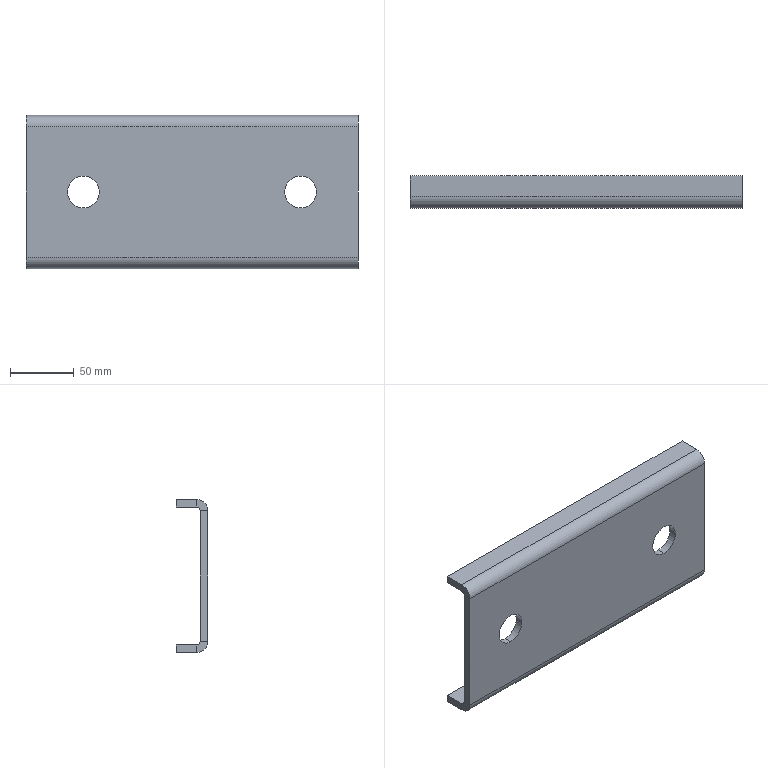Component | SolidWorks | THK-A1018FrontGuideWheelMountingPlate-1 | 1 solid | 26 faces | box 260 x 25 x 120 mm | volume 232555 mm3 | plane 18 | cylinder 8 | commonest cylinder face diameters 25 x4 18 x2 6 x2 | material Q235A
STEP:
#1=CARTESIAN_POINT('',(3.346,-5.079,-46.004));
#2=VERTEX_POINT('',#1);
#3=CARTESIAN_POINT('',(3.346,-5.079,-46.988));
#4=VERTEX_POINT('',#3);
#5=CARTESIAN_POINT('',(3.346,-5.079,-46.496));
#6=DIRECTION('',(0.,-1.,0.));
#7=DIRECTION('',(0.,0.,-1.));
#8=AXIS2_PLACEMENT_3D('',#5,#6,#7);
#9=CIRCLE('',#8,0.4921);
#10=EDGE_CURVE('',#2,#4,#9,.T.);
#11=ORIENTED_EDGE('',*,*,#10,.F.);
#12=CARTESIAN_POINT('',(3.346,-5.315,-46.004));
#13=VERTEX_POINT('',#12);
#14=CARTESIAN_POINT('',(3.346,-5.315,-46.004));
#15=DIRECTION('',(0.,-1.,0.));
#16=VECTOR('',#15,39.37);
#17=LINE('',#14,#16);
#18=EDGE_CURVE('',#2,#13,#17,.T.);
#19=ORIENTED_EDGE('',*,*,#18,.T.);
#20=CARTESIAN_POINT('',(3.346,-5.315,-46.988));
#21=VERTEX_POINT('',#20);
#22=CARTESIAN_POINT('',(3.346,-5.315,-46.496));
#23=DIRECTION('',(0.,-1.,0.));
#24=DIRECTION('',(0.,0.,-1.));
#25=AXIS2_PLACEMENT_3D('',#22,#23,#24);
#26=CIRCLE('',#25,0.4921);
#27=EDGE_CURVE('',#13,#21,#26,.T.);
#28=ORIENTED_EDGE('',*,*,#27,.T.);
#29=CARTESIAN_POINT('',(3.346,-5.315,-46.988));
#30=DIRECTION('',(0.,-1.,0.));
#31=VECTOR('',#30,39.37);
#32=LINE('',#29,#31);
#33=EDGE_CURVE('',#4,#21,#32,.T.);
#34=ORIENTED_EDGE('',*,*,#33,.F.);
#35=EDGE_LOOP('',(#11,#19,#28,#34));
#36=FACE_OUTER_BOUND('',#35,.T.);
#37=CARTESIAN_POINT('',(3.346,-5.315,-46.496));
#38=DIRECTION('',(0.,-1.,0.));
#39=DIRECTION('',(0.,0.,-1.));
#40=AXIS2_PLACEMENT_3D('',#37,#38,#39);
#41=CYLINDRICAL_SURFACE('',#40,0.4921);
#42=ADVANCED_FACE('',(#36),#41,.F.);
#43=CARTESIAN_POINT('',(-3.346,-5.079,-46.004));
#44=VERTEX_POINT('',#43);
#45=CARTESIAN_POINT('',(-3.346,-5.079,-46.988));
#46=VERTEX_POINT('',#45);
#47=CARTESIAN_POINT('',(-3.346,-5.079,-46.496));
#48=DIRECTION('',(0.,-1.,0.));
#49=DIRECTION('',(0.,0.,-1.));
#50=AXIS2_PLACEMENT_3D('',#47,#48,#49);
#51=CIRCLE('',#50,0.4921);
#52=EDGE_CURVE('',#44,#46,#51,.T.);
#53=ORIENTED_EDGE('',*,*,#52,.F.);
#54=CARTESIAN_POINT('',(-3.346,-5.315,-46.004));
#55=VERTEX_POINT('',#54);
#56=CARTESIAN_POINT('',(-3.346,-5.315,-46.004));
#57=DIRECTION('',(0.,-1.,0.));
#58=VECTOR('',#57,39.37);
#59=LINE('',#56,#58);
#60=EDGE_CURVE('',#44,#55,#59,.T.);
#61=ORIENTED_EDGE('',*,*,#60,.T.);
#62=CARTESIAN_POINT('',(-3.346,-5.315,-46.988));
#63=VERTEX_POINT('',#62);
#64=CARTESIAN_POINT('',(-3.346,-5.315,-46.496));
#65=DIRECTION('',(0.,-1.,0.));
#66=DIRECTION('',(0.,0.,-1.));
#67=AXIS2_PLACEMENT_3D('',#64,#65,#66);
#68=CIRCLE('',#67,0.4921);
#69=EDGE_CURVE('',#55,#63,#68,.T.);
#70=ORIENTED_EDGE('',*,*,#69,.T.);
#71=CARTESIAN_POINT('',(-3.346,-5.315,-46.988));
#72=DIRECTION('',(0.,-1.,0.));
#73=VECTOR('',#72,39.37);
#74=LINE('',#71,#73);
#75=EDGE_CURVE('',#46,#63,#74,.T.);
#76=ORIENTED_EDGE('',*,*,#75,.F.);
#77=EDGE_LOOP('',(#53,#61,#70,#76));
#78=FACE_OUTER_BOUND('',#77,.T.);
#79=CARTESIAN_POINT('',(-3.346,-5.315,-46.496));
#80=DIRECTION('',(0.,-1.,0.));
#81=DIRECTION('',(0.,0.,-1.));
#82=AXIS2_PLACEMENT_3D('',#79,#80,#81);
#83=CYLINDRICAL_SURFACE('',#82,0.4921);
#84=ADVANCED_FACE('',(#78),#83,.F.);
#85=CARTESIAN_POINT('',(5.118,-5.315,-48.504));
#86=VERTEX_POINT('',#85);
#87=CARTESIAN_POINT('',(5.118,-5.079,-48.504));
#88=VERTEX_POINT('',#87);
#89=CARTESIAN_POINT('',(5.118,-5.315,-48.504));
#90=DIRECTION('',(0.,1.,0.));
#91=VECTOR('',#90,39.37);
#92=LINE('',#89,#91);
#93=EDGE_CURVE('',#86,#88,#92,.T.);
#94=ORIENTED_EDGE('',*,*,#93,.F.);
#95=CARTESIAN_POINT('',(5.118,-4.961,-48.858));
#96=VERTEX_POINT('',#95);
#97=CARTESIAN_POINT('',(5.118,-4.961,-48.504));
#98=DIRECTION('',(-1.,0.,0.));
#99=DIRECTION('',(0.,0.,-1.));
#100=AXIS2_PLACEMENT_3D('',#97,#98,#99);
#101=CIRCLE('',#100,0.3543);
#102=EDGE_CURVE('',#96,#86,#101,.T.);
#103=ORIENTED_EDGE('',*,*,#102,.F.);
#104=CARTESIAN_POINT('',(5.118,-4.961,-48.622));
#105=VERTEX_POINT('',#104);
#106=CARTESIAN_POINT('',(5.118,-4.961,-48.622));
#107=DIRECTION('',(0.,0.,-1.));
#108=VECTOR('',#107,39.37);
#109=LINE('',#106,#108);
#110=EDGE_CURVE('',#105,#96,#109,.T.);
#111=ORIENTED_EDGE('',*,*,#110,.F.);
#112=CARTESIAN_POINT('',(5.118,-4.961,-48.504));
#113=DIRECTION('',(-1.,0.,0.));
#114=DIRECTION('',(0.,0.,-1.));
#115=AXIS2_PLACEMENT_3D('',#112,#113,#114);
#116=CIRCLE('',#115,0.1181);
#117=EDGE_CURVE('',#105,#88,#116,.T.);
#118=ORIENTED_EDGE('',*,*,#117,.T.);
#119=EDGE_LOOP('',(#94,#103,#111,#118));
#120=FACE_OUTER_BOUND('',#119,.T.);
#121=CARTESIAN_POINT('',(5.118,-5.315,-48.504));
#122=DIRECTION('',(1.,0.,0.));
#123=DIRECTION('',(0.,0.,-1.));
#124=AXIS2_PLACEMENT_3D('',#121,#122,#123);
#125=PLANE('',#124);
#126=ADVANCED_FACE('',(#120),#125,.T.);
#127=CARTESIAN_POINT('',(5.118,-5.315,-44.488));
#128=VERTEX_POINT('',#127);
#129=CARTESIAN_POINT('',(5.118,-5.315,-44.134));
#130=DIRECTION('',(0.,0.,1.));
#131=VECTOR('',#130,39.37);
#132=LINE('',#129,#131);
#133=EDGE_CURVE('',#86,#128,#132,.T.);
#134=ORIENTED_EDGE('',*,*,#133,.F.);
#135=ORIENTED_EDGE('',*,*,#93,.T.);
#136=CARTESIAN_POINT('',(5.118,-5.079,-44.488));
#137=VERTEX_POINT('',#136);
#138=CARTESIAN_POINT('',(5.118,-5.079,-44.134));
#139=DIRECTION('',(0.,0.,1.));
#140=VECTOR('',#139,39.37);
#141=LINE('',#138,#140);
#142=EDGE_CURVE('',#88,#137,#141,.T.);
#143=ORIENTED_EDGE('',*,*,#142,.T.);
#144=CARTESIAN_POINT('',(5.118,-5.079,-44.488));
#145=DIRECTION('',(0.,-1.,0.));
#146=VECTOR('',#145,39.37);
#147=LINE('',#144,#146);
#148=EDGE_CURVE('',#137,#128,#147,.T.);
#149=ORIENTED_EDGE('',*,*,#148,.T.);
#150=EDGE_LOOP('',(#134,#135,#143,#149));
#151=FACE_OUTER_BOUND('',#150,.T.);
#152=CARTESIAN_POINT('',(5.118,-4.961,-48.622));
#153=DIRECTION('',(1.,0.,0.));
#154=DIRECTION('',(0.,0.,-1.));
#155=AXIS2_PLACEMENT_3D('',#152,#153,#154);
#156=PLANE('',#155);
#157=ADVANCED_FACE('',(#151),#156,.T.);
#158=CARTESIAN_POINT('',(-5.118,-4.961,-48.858));
#159=VERTEX_POINT('',#158);
#160=CARTESIAN_POINT('',(-5.118,-4.961,-48.622));
#161=VERTEX_POINT('',#160);
#162=CARTESIAN_POINT('',(-5.118,-4.961,-48.858));
#163=DIRECTION('',(0.,0.,1.));
#164=VECTOR('',#163,39.37);
#165=LINE('',#162,#164);
#166=EDGE_CURVE('',#159,#161,#165,.T.);
#167=ORIENTED_EDGE('',*,*,#166,.F.);
#168=CARTESIAN_POINT('',(-5.118,-5.315,-48.504));
#169=VERTEX_POINT('',#168);
#170=CARTESIAN_POINT('',(-5.118,-4.961,-48.504));
#171=DIRECTION('',(-1.,0.,0.));
#172=DIRECTION('',(0.,0.,-1.));
#173=AXIS2_PLACEMENT_3D('',#170,#171,#172);
#174=CIRCLE('',#173,0.3543);
#175=EDGE_CURVE('',#159,#169,#174,.T.);
#176=ORIENTED_EDGE('',*,*,#175,.T.);
#177=CARTESIAN_POINT('',(-5.118,-5.079,-48.504));
#178=VERTEX_POINT('',#177);
#179=CARTESIAN_POINT('',(-5.118,-5.079,-48.504));
#180=DIRECTION('',(0.,-1.,0.));
#181=VECTOR('',#180,39.37);
#182=LINE('',#179,#181);
#183=EDGE_CURVE('',#178,#169,#182,.T.);
#184=ORIENTED_EDGE('',*,*,#183,.F.);
#185=CARTESIAN_POINT('',(-5.118,-4.961,-48.504));
#186=DIRECTION('',(-1.,0.,0.));
#187=DIRECTION('',(0.,0.,-1.));
#188=AXIS2_PLACEMENT_3D('',#185,#186,#187);
#189=CIRCLE('',#188,0.1181);
#190=EDGE_CURVE('',#161,#178,#189,.T.);
#191=ORIENTED_EDGE('',*,*,#190,.F.);
#192=EDGE_LOOP('',(#167,#176,#184,#191));
#193=FACE_OUTER_BOUND('',#192,.T.);
#194=CARTESIAN_POINT('',(-5.118,-4.961,-48.858));
#195=DIRECTION('',(-1.,0.,0.));
#196=DIRECTION('',(0.,0.,1.));
#197=AXIS2_PLACEMENT_3D('',#194,#195,#196);
#198=PLANE('',#197);
#199=ADVANCED_FACE('',(#193),#198,.T.);
#200=CARTESIAN_POINT('',(-5.118,-4.331,-48.858));
#201=VERTEX_POINT('',#200);
#202=CARTESIAN_POINT('',(-5.118,-5.315,-48.858));
#203=DIRECTION('',(0.,-1.,0.));
#204=VECTOR('',#203,39.37);
#205=LINE('',#202,#204);
#206=EDGE_CURVE('',#201,#159,#205,.T.);
#207=ORIENTED_EDGE('',*,*,#206,.T.);
#208=ORIENTED_EDGE('',*,*,#166,.T.);
#209=CARTESIAN_POINT('',(-5.118,-4.331,-48.622));
#210=VERTEX_POINT('',#209);
#211=CARTESIAN_POINT('',(-5.118,-5.315,-48.622));
#212=DIRECTION('',(0.,-1.,0.));
#213=VECTOR('',#212,39.37);
#214=LINE('',#211,#213);
#215=EDGE_CURVE('',#210,#161,#214,.T.);
#216=ORIENTED_EDGE('',*,*,#215,.F.);
#217=CARTESIAN_POINT('',(-5.118,-4.331,-48.622));
#218=DIRECTION('',(0.,0.,-1.));
#219=VECTOR('',#218,39.37);
#220=LINE('',#217,#219);
#221=EDGE_CURVE('',#210,#201,#220,.T.);
#222=ORIENTED_EDGE('',*,*,#221,.T.);
#223=EDGE_LOOP('',(#207,#208,#216,#222));
#224=FACE_OUTER_BOUND('',#223,.T.);
#225=CARTESIAN_POINT('',(-5.118,-5.079,-48.504));
#226=DIRECTION('',(-1.,0.,0.));
#227=DIRECTION('',(0.,0.,1.));
#228=AXIS2_PLACEMENT_3D('',#225,#226,#227);
#229=PLANE('',#228);
#230=ADVANCED_FACE('',(#224),#229,.T.);
#231=CARTESIAN_POINT('',(5.118,-4.961,-44.134));
#232=VERTEX_POINT('',#231);
#233=CARTESIAN_POINT('',(5.118,-4.961,-44.37));
#234=VERTEX_POINT('',#233);
#235=CARTESIAN_POINT('',(5.118,-4.961,-44.134));
#236=DIRECTION('',(0.,0.,-1.));
#237=VECTOR('',#236,39.37);
#238=LINE('',#235,#237);
#239=EDGE_CURVE('',#232,#234,#238,.T.);
#240=ORIENTED_EDGE('',*,*,#239,.F.);
#241=CARTESIAN_POINT('',(5.118,-4.961,-44.488));
#242=DIRECTION('',(-1.,0.,0.));
#243=DIRECTION('',(0.,0.,-1.));
#244=AXIS2_PLACEMENT_3D('',#241,#242,#243);
#245=CIRCLE('',#244,0.3543);
#246=EDGE_CURVE('',#128,#232,#245,.T.);
#247=ORIENTED_EDGE('',*,*,#246,.F.);
#248=ORIENTED_EDGE('',*,*,#148,.F.);
#249=CARTESIAN_POINT('',(5.118,-4.961,-44.488));
#250=DIRECTION('',(-1.,0.,0.));
#251=DIRECTION('',(0.,0.,-1.));
#252=AXIS2_PLACEMENT_3D('',#249,#250,#251);
#253=CIRCLE('',#252,0.1181);
#254=EDGE_CURVE('',#137,#234,#253,.T.);
#255=ORIENTED_EDGE('',*,*,#254,.T.);
#256=EDGE_LOOP('',(#240,#247,#248,#255));
#257=FACE_OUTER_BOUND('',#256,.T.);
#258=CARTESIAN_POINT('',(5.118,-4.961,-44.134));
#259=DIRECTION('',(1.,0.,0.));
#260=DIRECTION('',(0.,0.,-1.));
#261=AXIS2_PLACEMENT_3D('',#258,#259,#260);
#262=PLANE('',#261);
#263=ADVANCED_FACE('',(#257),#262,.T.);
#264=CARTESIAN_POINT('',(5.118,-4.331,-44.134));
#265=VERTEX_POINT('',#264);
#266=CARTESIAN_POINT('',(5.118,-5.315,-44.134));
#267=DIRECTION('',(0.,1.,0.));
#268=VECTOR('',#267,39.37);
#269=LINE('',#266,#268);
#270=EDGE_CURVE('',#232,#265,#269,.T.);
#271=ORIENTED_EDGE('',*,*,#270,.F.);
#272=ORIENTED_EDGE('',*,*,#239,.T.);
#273=CARTESIAN_POINT('',(5.118,-4.331,-44.37));
#274=VERTEX_POINT('',#273);
#275=CARTESIAN_POINT('',(5.118,-5.315,-44.37));
#276=DIRECTION('',(0.,1.,0.));
#277=VECTOR('',#276,39.37);
#278=LINE('',#275,#277);
#279=EDGE_CURVE('',#234,#274,#278,.T.);
#280=ORIENTED_EDGE('',*,*,#279,.T.);
#281=CARTESIAN_POINT('',(5.118,-4.331,-44.134));
#282=DIRECTION('',(0.,0.,-1.));
#283=VECTOR('',#282,39.37);
#284=LINE('',#281,#283);
#285=EDGE_CURVE('',#265,#274,#284,.T.);
#286=ORIENTED_EDGE('',*,*,#285,.F.);
#287=EDGE_LOOP('',(#271,#272,#280,#286));
#288=FACE_OUTER_BOUND('',#287,.T.);
#289=CARTESIAN_POINT('',(5.118,-5.079,-44.488));
#290=DIRECTION('',(1.,0.,0.));
#291=DIRECTION('',(0.,0.,-1.));
#292=AXIS2_PLACEMENT_3D('',#289,#290,#291);
#293=PLANE('',#292);
#294=ADVANCED_FACE('',(#288),#293,.T.);
#295=CARTESIAN_POINT('',(-5.118,-5.315,-44.488));
#296=VERTEX_POINT('',#295);
#297=CARTESIAN_POINT('',(-5.118,-5.079,-44.488));
#298=VERTEX_POINT('',#297);
#299=CARTESIAN_POINT('',(-5.118,-5.315,-44.488));
#300=DIRECTION('',(0.,1.,0.));
#301=VECTOR('',#300,39.37);
#302=LINE('',#299,#301);
#303=EDGE_CURVE('',#296,#298,#302,.T.);
#304=ORIENTED_EDGE('',*,*,#303,.F.);
#305=CARTESIAN_POINT('',(-5.118,-4.961,-44.134));
#306=VERTEX_POINT('',#305);
#307=CARTESIAN_POINT('',(-5.118,-4.961,-44.488));
#308=DIRECTION('',(-1.,0.,0.));
#309=DIRECTION('',(0.,0.,-1.));
#310=AXIS2_PLACEMENT_3D('',#307,#308,#309);
#311=CIRCLE('',#310,0.3543);
#312=EDGE_CURVE('',#296,#306,#311,.T.);
#313=ORIENTED_EDGE('',*,*,#312,.T.);
#314=CARTESIAN_POINT('',(-5.118,-4.961,-44.37));
#315=VERTEX_POINT('',#314);
#316=CARTESIAN_POINT('',(-5.118,-4.961,-44.37));
#317=DIRECTION('',(0.,0.,1.));
#318=VECTOR('',#317,39.37);
#319=LINE('',#316,#318);
#320=EDGE_CURVE('',#315,#306,#319,.T.);
#321=ORIENTED_EDGE('',*,*,#320,.F.);
#322=CARTESIAN_POINT('',(-5.118,-4.961,-44.488));
#323=DIRECTION('',(-1.,0.,0.));
#324=DIRECTION('',(0.,0.,-1.));
#325=AXIS2_PLACEMENT_3D('',#322,#323,#324);
#326=CIRCLE('',#325,0.1181);
#327=EDGE_CURVE('',#298,#315,#326,.T.);
#328=ORIENTED_EDGE('',*,*,#327,.F.);
#329=EDGE_LOOP('',(#304,#313,#321,#328));
#330=FACE_OUTER_BOUND('',#329,.T.);
#331=CARTESIAN_POINT('',(-5.118,-5.315,-44.488));
#332=DIRECTION('',(-1.,0.,0.));
#333=DIRECTION('',(0.,0.,1.));
#334=AXIS2_PLACEMENT_3D('',#331,#332,#333);
#335=PLANE('',#334);
#336=ADVANCED_FACE('',(#330),#335,.T.);
#337=CARTESIAN_POINT('',(-5.118,-5.315,-44.134));
#338=DIRECTION('',(0.,0.,1.));
#339=VECTOR('',#338,39.37);
#340=LINE('',#337,#339);
#341=EDGE_CURVE('',#169,#296,#340,.T.);
#342=ORIENTED_EDGE('',*,*,#341,.T.);
#343=ORIENTED_EDGE('',*,*,#303,.T.);
#344=CARTESIAN_POINT('',(-5.118,-5.079,-44.134));
#345=DIRECTION('',(0.,0.,1.));
#346=VECTOR('',#345,39.37);
#347=LINE('',#344,#346);
#348=EDGE_CURVE('',#178,#298,#347,.T.);
#349=ORIENTED_EDGE('',*,*,#348,.F.);
#350=ORIENTED_EDGE('',*,*,#183,.T.);
#351=EDGE_LOOP('',(#342,#343,#349,#350));
#352=FACE_OUTER_BOUND('',#351,.T.);
#353=CARTESIAN_POINT('',(-5.118,-4.961,-44.37));
#354=DIRECTION('',(-1.,0.,0.));
#355=DIRECTION('',(0.,0.,1.));
#356=AXIS2_PLACEMENT_3D('',#353,#354,#355);
#357=PLANE('',#356);
#358=ADVANCED_FACE('',(#352),#357,.T.);
#359=CARTESIAN_POINT('',(-5.118,-4.331,-44.37));
#360=VERTEX_POINT('',#359);
#361=CARTESIAN_POINT('',(-5.118,-5.315,-44.37));
#362=DIRECTION('',(0.,1.,0.));
#363=VECTOR('',#362,39.37);
#364=LINE('',#361,#363);
#365=EDGE_CURVE('',#315,#360,#364,.T.);
#366=ORIENTED_EDGE('',*,*,#365,.T.);
#367=CARTESIAN_POINT('',(5.118,-4.331,-44.37));
#368=DIRECTION('',(-1.,0.,0.));
#369=VECTOR('',#368,39.37);
#370=LINE('',#367,#369);
#371=EDGE_CURVE('',#274,#360,#370,.T.);
#372=ORIENTED_EDGE('',*,*,#371,.F.);
#373=ORIENTED_EDGE('',*,*,#279,.F.);
#374=CARTESIAN_POINT('',(5.118,-4.961,-44.37));
#375=DIRECTION('',(-1.,0.,0.));
#376=VECTOR('',#375,39.37);
#377=LINE('',#374,#376);
#378=EDGE_CURVE('',#234,#315,#377,.T.);
#379=ORIENTED_EDGE('',*,*,#378,.T.);
#380=EDGE_LOOP('',(#366,#372,#373,#379));
#381=FACE_OUTER_BOUND('',#380,.T.);
#382=CARTESIAN_POINT('',(5.118,-5.315,-44.37));
#383=DIRECTION('',(0.,0.,1.));
#384=DIRECTION('',(1.,0.,0.));
#385=AXIS2_PLACEMENT_3D('',#382,#383,#384);
#386=PLANE('',#385);
#387=ADVANCED_FACE('',(#381),#386,.F.);
#388=CARTESIAN_POINT('',(-5.118,-4.331,-44.134));
#389=VERTEX_POINT('',#388);
#390=CARTESIAN_POINT('',(-5.118,-4.331,-44.134));
#391=DIRECTION('',(0.,0.,-1.));
#392=VECTOR('',#391,39.37);
#393=LINE('',#390,#392);
#394=EDGE_CURVE('',#389,#360,#393,.T.);
#395=ORIENTED_EDGE('',*,*,#394,.F.);
#396=CARTESIAN_POINT('',(5.118,-4.331,-44.134));
#397=DIRECTION('',(-1.,0.,0.));
#398=VECTOR('',#397,39.37);
#399=LINE('',#396,#398);
#400=EDGE_CURVE('',#265,#389,#399,.T.);
#401=ORIENTED_EDGE('',*,*,#400,.F.);
#402=ORIENTED_EDGE('',*,*,#285,.T.);
#403=ORIENTED_EDGE('',*,*,#371,.T.);
#404=EDGE_LOOP('',(#395,#401,#402,#403));
#405=FACE_OUTER_BOUND('',#404,.T.);
#406=CARTESIAN_POINT('',(5.118,-4.331,-44.134));
#407=DIRECTION('',(0.,1.,0.));
#408=DIRECTION('',(0.,0.,1.));
#409=AXIS2_PLACEMENT_3D('',#406,#407,#408);
#410=PLANE('',#409);
#411=ADVANCED_FACE('',(#405),#410,.T.);
#412=CARTESIAN_POINT('',(-5.118,-5.315,-44.134));
#413=DIRECTION('',(0.,1.,0.));
#414=VECTOR('',#413,39.37);
#415=LINE('',#412,#414);
#416=EDGE_CURVE('',#306,#389,#415,.T.);
#417=ORIENTED_EDGE('',*,*,#416,.F.);
#418=CARTESIAN_POINT('',(5.118,-4.961,-44.134));
#419=DIRECTION('',(-1.,0.,0.));
#420=VECTOR('',#419,39.37);
#421=LINE('',#418,#420);
#422=EDGE_CURVE('',#232,#306,#421,.T.);
#423=ORIENTED_EDGE('',*,*,#422,.F.);
#424=ORIENTED_EDGE('',*,*,#270,.T.);
#425=ORIENTED_EDGE('',*,*,#400,.T.);
#426=EDGE_LOOP('',(#417,#423,#424,#425));
#427=FACE_OUTER_BOUND('',#426,.T.);
#428=CARTESIAN_POINT('',(5.118,-5.315,-44.134));
#429=DIRECTION('',(0.,0.,1.));
#430=DIRECTION('',(1.,0.,0.));
#431=AXIS2_PLACEMENT_3D('',#428,#429,#430);
#432=PLANE('',#431);
#433=ADVANCED_FACE('',(#427),#432,.T.);
#434=ORIENTED_EDGE('',*,*,#312,.F.);
#435=CARTESIAN_POINT('',(5.118,-5.315,-44.488));
#436=DIRECTION('',(-1.,0.,0.));
#437=VECTOR('',#436,39.37);
#438=LINE('',#435,#437);
#439=EDGE_CURVE('',#128,#296,#438,.T.);
#440=ORIENTED_EDGE('',*,*,#439,.F.);
#441=ORIENTED_EDGE('',*,*,#246,.T.);
#442=ORIENTED_EDGE('',*,*,#422,.T.);
#443=EDGE_LOOP('',(#434,#440,#441,#442));
#444=FACE_OUTER_BOUND('',#443,.T.);
#445=CARTESIAN_POINT('',(5.118,-4.961,-44.488));
#446=DIRECTION('',(-1.,0.,0.));
#447=DIRECTION('',(0.,0.,1.));
#448=AXIS2_PLACEMENT_3D('',#445,#446,#447);
#449=CYLINDRICAL_SURFACE('',#448,0.3543);
#450=ADVANCED_FACE('',(#444),#449,.T.);
#451=CARTESIAN_POINT('',(3.346,-5.315,-46.496));
#452=DIRECTION('',(0.,-1.,0.));
#453=DIRECTION('',(0.,0.,-1.));
#454=AXIS2_PLACEMENT_3D('',#451,#452,#453);
#455=CIRCLE('',#454,0.4921);
#456=EDGE_CURVE('',#21,#13,#455,.T.);
#457=ORIENTED_EDGE('',*,*,#456,.F.);
#458=ORIENTED_EDGE('',*,*,#27,.F.);
#459=EDGE_LOOP('',(#457,#458));
#460=FACE_BOUND('',#459,.T.);
#461=CARTESIAN_POINT('',(-3.346,-5.315,-46.496));
#462=DIRECTION('',(0.,-1.,0.));
#463=DIRECTION('',(0.,0.,-1.));
#464=AXIS2_PLACEMENT_3D('',#461,#462,#463);
#465=CIRCLE('',#464,0.4921);
#466=EDGE_CURVE('',#63,#55,#465,.T.);
#467=ORIENTED_EDGE('',*,*,#466,.F.);
#468=ORIENTED_EDGE('',*,*,#69,.F.);
#469=EDGE_LOOP('',(#467,#468));
#470=FACE_BOUND('',#469,.T.);
#471=ORIENTED_EDGE('',*,*,#341,.F.);
#472=CARTESIAN_POINT('',(5.118,-5.315,-48.504));
#473=DIRECTION('',(-1.,0.,0.));
#474=VECTOR('',#473,39.37);
#475=LINE('',#472,#474);
#476=EDGE_CURVE('',#86,#169,#475,.T.);
#477=ORIENTED_EDGE('',*,*,#476,.F.);
#478=ORIENTED_EDGE('',*,*,#133,.T.);
#479=ORIENTED_EDGE('',*,*,#439,.T.);
#480=EDGE_LOOP('',(#471,#477,#478,#479));
#481=FACE_OUTER_BOUND('',#480,.T.);
#482=CARTESIAN_POINT('',(5.118,-5.315,-44.134));
#483=DIRECTION('',(0.,-1.,0.));
#484=DIRECTION('',(0.,0.,-1.));
#485=AXIS2_PLACEMENT_3D('',#482,#483,#484);
#486=PLANE('',#485);
#487=ADVANCED_FACE('',(#460,#470,#481),#486,.T.);
#488=ORIENTED_EDGE('',*,*,#175,.F.);
#489=CARTESIAN_POINT('',(5.118,-4.961,-48.858));
#490=DIRECTION('',(-1.,0.,0.));
#491=VECTOR('',#490,39.37);
#492=LINE('',#489,#491);
#493=EDGE_CURVE('',#96,#159,#492,.T.);
#494=ORIENTED_EDGE('',*,*,#493,.F.);
#495=ORIENTED_EDGE('',*,*,#102,.T.);
#496=ORIENTED_EDGE('',*,*,#476,.T.);
#497=EDGE_LOOP('',(#488,#494,#495,#496));
#498=FACE_OUTER_BOUND('',#497,.T.);
#499=CARTESIAN_POINT('',(5.118,-4.961,-48.504));
#500=DIRECTION('',(-1.,0.,0.));
#501=DIRECTION('',(0.,0.,1.));
#502=AXIS2_PLACEMENT_3D('',#499,#500,#501);
#503=CYLINDRICAL_SURFACE('',#502,0.3543);
#504=ADVANCED_FACE('',(#498),#503,.T.);
#505=ORIENTED_EDGE('',*,*,#206,.F.);
#506=CARTESIAN_POINT('',(5.118,-4.331,-48.858));
#507=VERTEX_POINT('',#506);
#508=CARTESIAN_POINT('',(5.118,-4.331,-48.858));
#509=DIRECTION('',(-1.,0.,0.));
#510=VECTOR('',#509,39.37);
#511=LINE('',#508,#510);
#512=EDGE_CURVE('',#507,#201,#511,.T.);
#513=ORIENTED_EDGE('',*,*,#512,.F.);
#514=CARTESIAN_POINT('',(5.118,-5.315,-48.858));
#515=DIRECTION('',(0.,-1.,0.));
#516=VECTOR('',#515,39.37);
#517=LINE('',#514,#516);
#518=EDGE_CURVE('',#507,#96,#517,.T.);
#519=ORIENTED_EDGE('',*,*,#518,.T.);
#520=ORIENTED_EDGE('',*,*,#493,.T.);
#521=EDGE_LOOP('',(#505,#513,#519,#520));
#522=FACE_OUTER_BOUND('',#521,.T.);
#523=CARTESIAN_POINT('',(5.118,-5.315,-48.858));
#524=DIRECTION('',(0.,0.,-1.));
#525=DIRECTION('',(-1.,0.,0.));
#526=AXIS2_PLACEMENT_3D('',#523,#524,#525);
#527=PLANE('',#526);
#528=ADVANCED_FACE('',(#522),#527,.T.);
#529=ORIENTED_EDGE('',*,*,#221,.F.);
#530=CARTESIAN_POINT('',(5.118,-4.331,-48.622));
#531=VERTEX_POINT('',#530);
#532=CARTESIAN_POINT('',(5.118,-4.331,-48.622));
#533=DIRECTION('',(-1.,0.,0.));
#534=VECTOR('',#533,39.37);
#535=LINE('',#532,#534);
#536=EDGE_CURVE('',#531,#210,#535,.T.);
#537=ORIENTED_EDGE('',*,*,#536,.F.);
#538=CARTESIAN_POINT('',(5.118,-4.331,-48.622));
#539=DIRECTION('',(0.,0.,-1.));
#540=VECTOR('',#539,39.37);
#541=LINE('',#538,#540);
#542=EDGE_CURVE('',#531,#507,#541,.T.);
#543=ORIENTED_EDGE('',*,*,#542,.T.);
#544=ORIENTED_EDGE('',*,*,#512,.T.);
#545=EDGE_LOOP('',(#529,#537,#543,#544));
#546=FACE_OUTER_BOUND('',#545,.T.);
#547=CARTESIAN_POINT('',(5.118,-4.331,-48.622));
#548=DIRECTION('',(0.,1.,0.));
#549=DIRECTION('',(0.,0.,1.));
#550=AXIS2_PLACEMENT_3D('',#547,#548,#549);
#551=PLANE('',#550);
#552=ADVANCED_FACE('',(#546),#551,.T.);
#553=ORIENTED_EDGE('',*,*,#215,.T.);
#554=CARTESIAN_POINT('',(5.118,-4.961,-48.622));
#555=DIRECTION('',(-1.,0.,0.));
#556=VECTOR('',#555,39.37);
#557=LINE('',#554,#556);
#558=EDGE_CURVE('',#105,#161,#557,.T.);
#559=ORIENTED_EDGE('',*,*,#558,.F.);
#560=CARTESIAN_POINT('',(5.118,-5.315,-48.622));
#561=DIRECTION('',(0.,-1.,0.));
#562=VECTOR('',#561,39.37);
#563=LINE('',#560,#562);
#564=EDGE_CURVE('',#531,#105,#563,.T.);
#565=ORIENTED_EDGE('',*,*,#564,.F.);
#566=ORIENTED_EDGE('',*,*,#536,.T.);
#567=EDGE_LOOP('',(#553,#559,#565,#566));
#568=FACE_OUTER_BOUND('',#567,.T.);
#569=CARTESIAN_POINT('',(5.118,-5.315,-48.622));
#570=DIRECTION('',(0.,0.,-1.));
#571=DIRECTION('',(-1.,0.,0.));
#572=AXIS2_PLACEMENT_3D('',#569,#570,#571);
#573=PLANE('',#572);
#574=ADVANCED_FACE('',(#568),#573,.F.);
#575=ORIENTED_EDGE('',*,*,#190,.T.);
#576=CARTESIAN_POINT('',(5.118,-5.079,-48.504));
#577=DIRECTION('',(-1.,0.,0.));
#578=VECTOR('',#577,39.37);
#579=LINE('',#576,#578);
#580=EDGE_CURVE('',#88,#178,#579,.T.);
#581=ORIENTED_EDGE('',*,*,#580,.F.);
#582=ORIENTED_EDGE('',*,*,#117,.F.);
#583=ORIENTED_EDGE('',*,*,#558,.T.);
#584=EDGE_LOOP('',(#575,#581,#582,#583));
#585=FACE_OUTER_BOUND('',#584,.T.);
#586=CARTESIAN_POINT('',(5.118,-4.961,-48.504));
#587=DIRECTION('',(-1.,0.,0.));
#588=DIRECTION('',(0.,0.,1.));
#589=AXIS2_PLACEMENT_3D('',#586,#587,#588);
#590=CYLINDRICAL_SURFACE('',#589,0.1181);
#591=ADVANCED_FACE('',(#585),#590,.F.);
#592=CARTESIAN_POINT('',(3.346,-5.079,-46.496));
#593=DIRECTION('',(0.,-1.,0.));
#594=DIRECTION('',(0.,0.,-1.));
#595=AXIS2_PLACEMENT_3D('',#592,#593,#594);
#596=CIRCLE('',#595,0.4921);
#597=EDGE_CURVE('',#4,#2,#596,.T.);
#598=ORIENTED_EDGE('',*,*,#597,.T.);
#599=ORIENTED_EDGE('',*,*,#10,.T.);
#600=EDGE_LOOP('',(#598,#599));
#601=FACE_BOUND('',#600,.T.);
#602=CARTESIAN_POINT('',(-3.346,-5.079,-46.496));
#603=DIRECTION('',(0.,-1.,0.));
#604=DIRECTION('',(0.,0.,-1.));
#605=AXIS2_PLACEMENT_3D('',#602,#603,#604);
#606=CIRCLE('',#605,0.4921);
#607=EDGE_CURVE('',#46,#44,#606,.T.);
#608=ORIENTED_EDGE('',*,*,#607,.T.);
#609=ORIENTED_EDGE('',*,*,#52,.T.);
#610=EDGE_LOOP('',(#608,#609));
#611=FACE_BOUND('',#610,.T.);
#612=ORIENTED_EDGE('',*,*,#348,.T.);
#613=CARTESIAN_POINT('',(5.118,-5.079,-44.488));
#614=DIRECTION('',(-1.,0.,0.));
#615=VECTOR('',#614,39.37);
#616=LINE('',#613,#615);
#617=EDGE_CURVE('',#137,#298,#616,.T.);
#618=ORIENTED_EDGE('',*,*,#617,.F.);
#619=ORIENTED_EDGE('',*,*,#142,.F.);
#620=ORIENTED_EDGE('',*,*,#580,.T.);
#621=EDGE_LOOP('',(#612,#618,#619,#620));
#622=FACE_OUTER_BOUND('',#621,.T.);
#623=CARTESIAN_POINT('',(5.118,-5.079,-44.134));
#624=DIRECTION('',(0.,-1.,0.));
#625=DIRECTION('',(0.,0.,-1.));
#626=AXIS2_PLACEMENT_3D('',#623,#624,#625);
#627=PLANE('',#626);
#628=ADVANCED_FACE('',(#601,#611,#622),#627,.F.);
#629=ORIENTED_EDGE('',*,*,#327,.T.);
#630=ORIENTED_EDGE('',*,*,#378,.F.);
#631=ORIENTED_EDGE('',*,*,#254,.F.);
#632=ORIENTED_EDGE('',*,*,#617,.T.);
#633=EDGE_LOOP('',(#629,#630,#631,#632));
#634=FACE_OUTER_BOUND('',#633,.T.);
#635=CARTESIAN_POINT('',(5.118,-4.961,-44.488));
#636=DIRECTION('',(-1.,0.,0.));
#637=DIRECTION('',(0.,0.,1.));
#638=AXIS2_PLACEMENT_3D('',#635,#636,#637);
#639=CYLINDRICAL_SURFACE('',#638,0.1181);
#640=ADVANCED_FACE('',(#634),#639,.F.);
#641=ORIENTED_EDGE('',*,*,#564,.T.);
#642=ORIENTED_EDGE('',*,*,#110,.T.);
#643=ORIENTED_EDGE('',*,*,#518,.F.);
#644=ORIENTED_EDGE('',*,*,#542,.F.);
#645=EDGE_LOOP('',(#641,#642,#643,#644));
#646=FACE_OUTER_BOUND('',#645,.T.);
#647=CARTESIAN_POINT('',(5.118,-4.961,-44.488));
#648=DIRECTION('',(1.,0.,0.));
#649=DIRECTION('',(0.,0.,-1.));
#650=AXIS2_PLACEMENT_3D('',#647,#648,#649);
#651=PLANE('',#650);
#652=ADVANCED_FACE('',(#646),#651,.T.);
#653=ORIENTED_EDGE('',*,*,#365,.F.);
#654=ORIENTED_EDGE('',*,*,#320,.T.);
#655=ORIENTED_EDGE('',*,*,#416,.T.);
#656=ORIENTED_EDGE('',*,*,#394,.T.);
#657=EDGE_LOOP('',(#653,#654,#655,#656));
#658=FACE_OUTER_BOUND('',#657,.T.);
#659=CARTESIAN_POINT('',(-5.118,-4.961,-44.488));
#660=DIRECTION('',(1.,0.,0.));
#661=DIRECTION('',(0.,0.,-1.));
#662=AXIS2_PLACEMENT_3D('',#659,#660,#661);
#663=PLANE('',#662);
#664=ADVANCED_FACE('',(#658),#663,.F.);
#665=ORIENTED_EDGE('',*,*,#60,.F.);
#666=ORIENTED_EDGE('',*,*,#607,.F.);
#667=ORIENTED_EDGE('',*,*,#75,.T.);
#668=ORIENTED_EDGE('',*,*,#466,.T.);
#669=EDGE_LOOP('',(#665,#666,#667,#668));
#670=FACE_OUTER_BOUND('',#669,.T.);
#671=CARTESIAN_POINT('',(-3.346,-5.315,-46.496));
#672=DIRECTION('',(0.,-1.,0.));
#673=DIRECTION('',(0.,0.,-1.));
#674=AXIS2_PLACEMENT_3D('',#671,#672,#673);
#675=CYLINDRICAL_SURFACE('',#674,0.4921);
#676=ADVANCED_FACE('',(#670),#675,.F.);
#677=ORIENTED_EDGE('',*,*,#18,.F.);
#678=ORIENTED_EDGE('',*,*,#597,.F.);
#679=ORIENTED_EDGE('',*,*,#33,.T.);
#680=ORIENTED_EDGE('',*,*,#456,.T.);
#681=EDGE_LOOP('',(#677,#678,#679,#680));
#682=FACE_OUTER_BOUND('',#681,.T.);
#683=CARTESIAN_POINT('',(3.346,-5.315,-46.496));
#684=DIRECTION('',(0.,-1.,0.));
#685=DIRECTION('',(0.,0.,-1.));
#686=AXIS2_PLACEMENT_3D('',#683,#684,#685);
#687=CYLINDRICAL_SURFACE('',#686,0.4921);
#688=ADVANCED_FACE('',(#682),#687,.F.);
#689=CLOSED_SHELL('',(#42,#84,#126,#157,#199,#230,#263,#294,#336,#358,#387,#411,#433,#450,#487,#504,#528,#552,#574,#591,#628,#640,#652,#664,#676,#688));
#690=MANIFOLD_SOLID_BREP('',#689);
#691=CARTESIAN_POINT('',(0.,0.,0.));
#692=DIRECTION('',(0.,0.,1.));
#693=DIRECTION('',(1.,0.,0.));
#694=AXIS2_PLACEMENT_3D('',#691,#692,#693);
#695=(LENGTH_UNIT()NAMED_UNIT(*)SI_UNIT($,.METRE.));
#696=LENGTH_MEASURE_WITH_UNIT(LENGTH_MEASURE(0.0254),#695);
#697=DIMENSIONAL_EXPONENTS(1.,0.,0.,0.,0.,0.,0.);
#698=(CONVERSION_BASED_UNIT('',#696)LENGTH_UNIT()NAMED_UNIT(#697));
#699=UNCERTAINTY_MEASURE_WITH_UNIT(LENGTH_MEASURE(0.00001),#698,'','');
#700=(NAMED_UNIT(*)PLANE_ANGLE_UNIT()SI_UNIT($,.RADIAN.));
#701=(NAMED_UNIT(*)SI_UNIT($,.STERADIAN.)SOLID_ANGLE_UNIT());
#702=(GEOMETRIC_REPRESENTATION_CONTEXT(3)GLOBAL_UNCERTAINTY_ASSIGNED_CONTEXT((#699))GLOBAL_UNIT_ASSIGNED_CONTEXT((#698,#700,#701))REPRESENTATION_CONTEXT('',''));
#703=ADVANCED_BREP_SHAPE_REPRESENTATION('',(#690,#694),#702);
#704=COLOUR_RGB('',0.7922,0.8196,0.9333);
#705=FILL_AREA_STYLE_COLOUR('',#704);
#706=FILL_AREA_STYLE('',(#705));
#707=SURFACE_STYLE_FILL_AREA(#706);
#708=SURFACE_SIDE_STYLE('',(#707));
#709=SURFACE_STYLE_USAGE(.BOTH.,#708);
#710=PRESENTATION_STYLE_ASSIGNMENT((#709));
#711=STYLED_ITEM('',(#710),#690);
#712=PRESENTATION_LAYER_ASSIGNMENT('','',(#711));
#713=(LENGTH_UNIT()NAMED_UNIT(*)SI_UNIT($,.METRE.));
#714=LENGTH_MEASURE_WITH_UNIT(LENGTH_MEASURE(0.0254),#713);
#715=DIMENSIONAL_EXPONENTS(1.,0.,0.,0.,0.,0.,0.);
#716=(CONVERSION_BASED_UNIT('',#714)LENGTH_UNIT()NAMED_UNIT(#715));
#717=UNCERTAINTY_MEASURE_WITH_UNIT(LENGTH_MEASURE(0.00001),#716,'','');
#718=(NAMED_UNIT(*)PLANE_ANGLE_UNIT()SI_UNIT($,.RADIAN.));
#719=(NAMED_UNIT(*)SI_UNIT($,.STERADIAN.)SOLID_ANGLE_UNIT());
#720=(GEOMETRIC_REPRESENTATION_CONTEXT(3)GLOBAL_UNCERTAINTY_ASSIGNED_CONTEXT((#717))GLOBAL_UNIT_ASSIGNED_CONTEXT((#716,#718,#719))REPRESENTATION_CONTEXT('',''));
#721=MECHANICAL_DESIGN_GEOMETRIC_PRESENTATION_REPRESENTATION('',(#711),#720);